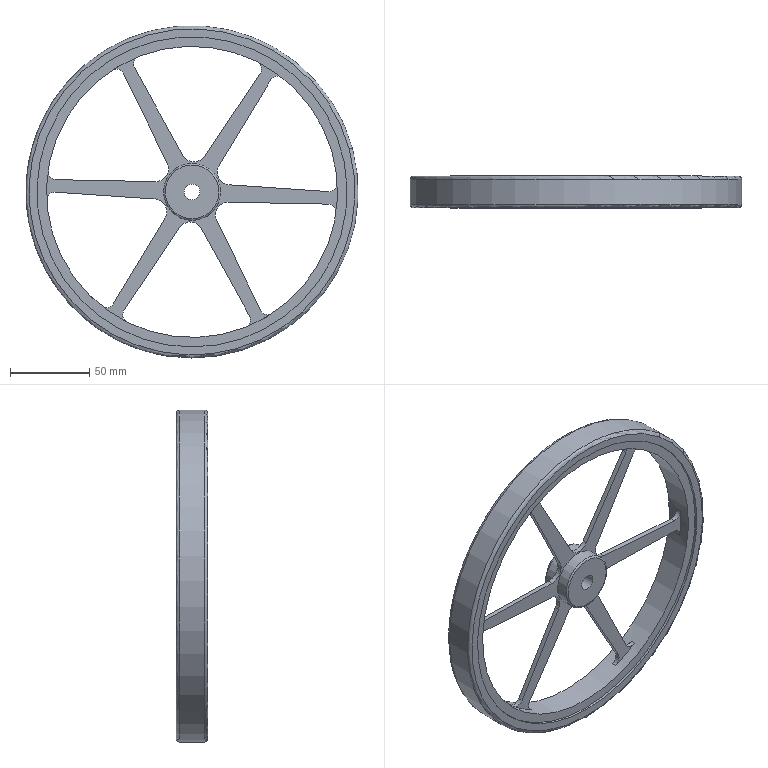Component | NX | BIG_FLYWHEEL | 1 solid | 49 faces | volume 180972 mm3 | cylinder 25 | plane 20 | torus 4 | commonest cylinder face diameters 10 x13 16 x6 196 x2 36 x2 210 x1 184 x1